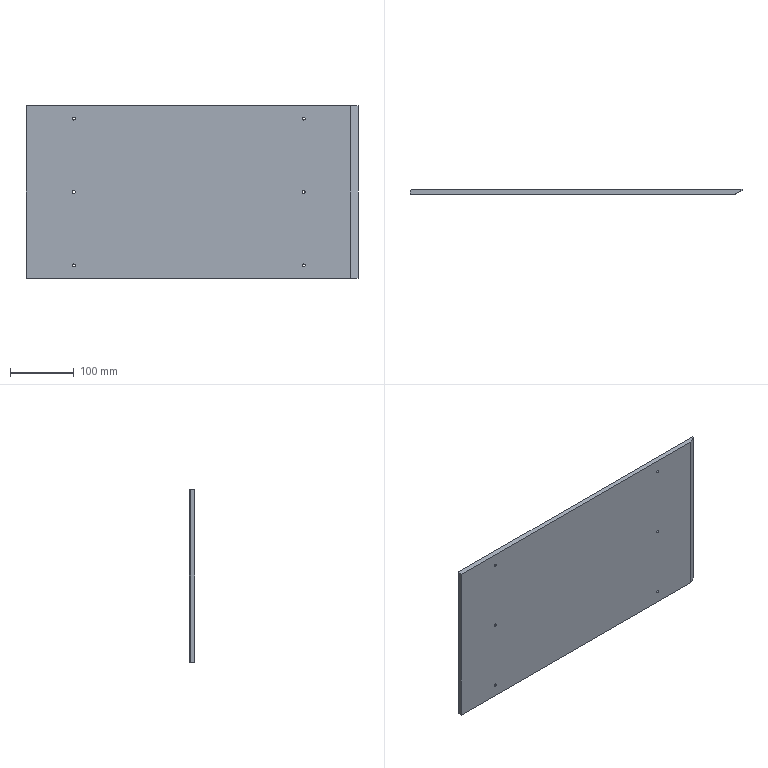Component | SolidWorks | LD101-02--Q1001-Q1-2-1 | 1 solid | 48 faces | box 520 x 8 x 270 mm | volume 1004018 mm3 | cylinder 24 | plane 24 | commonest cylinder face diameters 8 x12 4.5 x12 | material AL6061
build123d program:
from build123d import *

# Parameters (mm, degrees)
SKETCH1_W                                          = 520
SKETCH1_H                                          = 270
BOSS_EXTRUDE1_DEPTH                                = 4
CHAMFER1_SIZE                                      = 2
CUT_EXTRUDE1_DEPTH                                 = 375.855
HOLE_SIZE_FOR_HEX_SOCKET_HEAD_CAP_SCRE_D           = 4.5
HOLE_SIZE_FOR_HEX_SOCKET_HEAD_CAP_SCRE_CBORE_D     = 8
HOLE_SIZE_FOR_HEX_SOCKET_HEAD_CAP_SCRE_CBORE_DEPTH = 4.6
WEAR_STRIP_GROOVE_SKETCH_W                         = 40
WEAR_STRIP_GROOVE_SKETCH_H                         = 266
WEAR_STRIP_SLOT_DEPTH                              = 5


with BuildPart() as part:
    # Sketch1 → Boss-Extrude1 (new, symmetric)
    with BuildSketch(Plane(origin=(0, 0, 0), x_dir=(1, 0, 0), z_dir=(0, 1, 0))):
        Rectangle(SKETCH1_W, SKETCH1_H)
    extrude(amount=BOSS_EXTRUDE1_DEPTH, both=True)

    # Chamfer1
    chamfer1_edges = [part.edges().sort_by_distance(p)[0] for p in [
        (-260, 4, 0),
    ]]
    chamfer(chamfer1_edges, length=CHAMFER1_SIZE)

    # Sketch4 → Cut-Extrude1 (cut, through all)
    with BuildSketch(Plane.XY.offset(135)):
        Polygon((260, 2.5), (248, -4), (260, -4), align=None)
    extrude(amount=-CUT_EXTRUDE1_DEPTH, mode=Mode.SUBTRACT)

    # Hole Size _for_ Hex Socket Head Cap Scre (through all)
    with Locations(Plane(origin=(0, 4, 0), x_dir=(1, 0, 0), z_dir=(0, 1, 0))):
        with Locations((-185, 115), (-185, -115), (175, -115), (175, 115), (-185, 0), (175, 0)):
            CounterBoreHole(HOLE_SIZE_FOR_HEX_SOCKET_HEAD_CAP_SCRE_D / 2, HOLE_SIZE_FOR_HEX_SOCKET_HEAD_CAP_SCRE_CBORE_D / 2, HOLE_SIZE_FOR_HEX_SOCKET_HEAD_CAP_SCRE_CBORE_DEPTH)

    # Wear Strip Groove Sketch → Wear Strip Slot (cut)
    with BuildSketch(Plane(origin=(0, 4, 0), x_dir=(1, 0, 0), z_dir=(0, 1, 0))):
        with Locations((-230, 0)):
            Rectangle(WEAR_STRIP_GROOVE_SKETCH_W, WEAR_STRIP_GROOVE_SKETCH_H)
        with Locations((210, 0)):
            Rectangle(WEAR_STRIP_GROOVE_SKETCH_W, WEAR_STRIP_GROOVE_SKETCH_H)
    extrude(amount=-WEAR_STRIP_SLOT_DEPTH, mode=Mode.SUBTRACT)


solid = part.part

# Placed as in the assembly
solid = solid.moved(Location((-160.29, -152.897, 146.257), (0, 0, 0)))